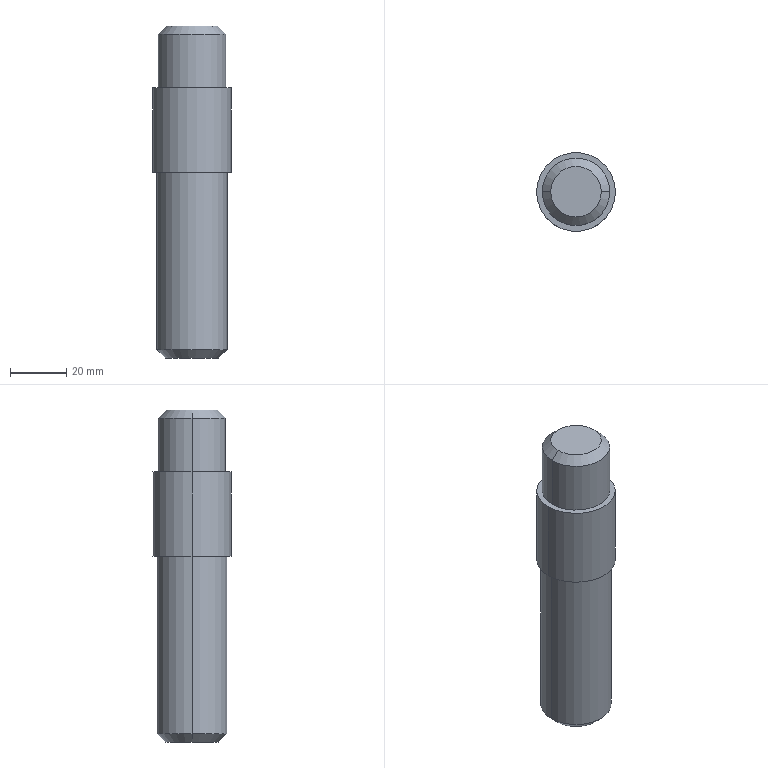Component | SolidWorks | PolishingAxis-1 | 1 solid | 14 faces | box 28 x 28 x 118 mm | volume 60187 mm3 | cylinder 6 | cone 4 | plane 4 | commonest cylinder face diameters 25 x2 24 x2 28 x2
build123d program:
from build123d import *

# Parameters (mm, degrees)
SKETCH1_R           = 12
BOSS_EXTRUDE1_DEPTH = 22
SKETCH2_R           = 14
BOSS_EXTRUDE2_DEPTH = 96
CUT_EXTRUDE1_START  = -66
SKETCH3_R           = 14
SKETCH3_R_2         = 12.5
CUT_EXTRUDE1_DEPTH  = 66
CHAMFER1_SIZE       = 3


with BuildPart() as part:
    # Sketch1 → Boss-Extrude1 (new body)
    with BuildSketch(Plane.XY):
        Circle(SKETCH1_R)
    extrude(amount=-BOSS_EXTRUDE1_DEPTH)

    # Sketch2 → Boss-Extrude2 (add)
    with BuildSketch(Plane.XY):
        Circle(SKETCH2_R)
    extrude(amount=BOSS_EXTRUDE2_DEPTH)

    # Sketch3 → Cut-Extrude1 (cut)
    with BuildSketch(Plane.XY.offset(96).offset(CUT_EXTRUDE1_START)):
        Circle(SKETCH3_R)
        Circle(SKETCH3_R_2, mode=Mode.SUBTRACT)
    extrude(amount=CUT_EXTRUDE1_DEPTH, mode=Mode.SUBTRACT)

    # Chamfer1
    chamfer1_edges = [part.edges().sort_by_distance(p)[0] for p in [
        (-12.5, 0, 96),
        (-12, 0, -22),
    ]]
    chamfer(chamfer1_edges, length=CHAMFER1_SIZE)


solid = part.part

# Placed as in the assembly
solid = solid.moved(Location((0, 0, -116), (180, 0, 0)))
STEP:
#1=COLOUR_RGB('',0.7922,0.8196,0.9333);
#2=FILL_AREA_STYLE_COLOUR('',#1);
#3=FILL_AREA_STYLE('',(#2));
#4=SURFACE_STYLE_FILL_AREA(#3);
#5=SURFACE_SIDE_STYLE('',(#4));
#6=SURFACE_STYLE_USAGE(.BOTH.,#5);
#7=PRESENTATION_STYLE_ASSIGNMENT((#6));
#8=CARTESIAN_POINT('',(-0.374,0.,-8.346));
#9=VERTEX_POINT('',#8);
#10=CARTESIAN_POINT('',(0.374,0.,-8.346));
#11=VERTEX_POINT('',#10);
#12=CARTESIAN_POINT('',(0.,0.,-8.346));
#13=DIRECTION('',(0.,0.,-1.));
#14=DIRECTION('',(-1.,0.,0.));
#15=AXIS2_PLACEMENT_3D('',#12,#13,#14);
#16=CIRCLE('',#15,0.374);
#17=EDGE_CURVE('',#9,#11,#16,.T.);
#18=ORIENTED_EDGE('',*,*,#17,.F.);
#19=CARTESIAN_POINT('',(-0.4921,0.,-8.228));
#20=VERTEX_POINT('',#19);
#21=CARTESIAN_POINT('',(-0.374,0.,-8.346));
#22=DIRECTION('',(-0.7071,0.,0.7071));
#23=VECTOR('',#22,39.37);
#24=LINE('',#21,#23);
#25=EDGE_CURVE('',#9,#20,#24,.T.);
#26=ORIENTED_EDGE('',*,*,#25,.T.);
#27=CARTESIAN_POINT('',(0.4921,0.,-8.228));
#28=VERTEX_POINT('',#27);
#29=CARTESIAN_POINT('',(0.,0.,-8.228));
#30=DIRECTION('',(0.,0.,1.));
#31=DIRECTION('',(-1.,0.,0.));
#32=AXIS2_PLACEMENT_3D('',#29,#30,#31);
#33=CIRCLE('',#32,0.4921);
#34=EDGE_CURVE('',#28,#20,#33,.T.);
#35=ORIENTED_EDGE('',*,*,#34,.F.);
#36=CARTESIAN_POINT('',(0.374,0.,-8.346));
#37=DIRECTION('',(0.7071,0.,0.7071));
#38=VECTOR('',#37,39.37);
#39=LINE('',#36,#38);
#40=EDGE_CURVE('',#11,#28,#39,.T.);
#41=ORIENTED_EDGE('',*,*,#40,.F.);
#42=EDGE_LOOP('',(#18,#26,#35,#41));
#43=FACE_OUTER_BOUND('',#42,.T.);
#44=CARTESIAN_POINT('',(0.,0.,-8.346));
#45=DIRECTION('',(0.,0.,1.));
#46=DIRECTION('',(1.,0.,0.));
#47=AXIS2_PLACEMENT_3D('',#44,#45,#46);
#48=CONICAL_SURFACE('',#47,0.374,0.7854);
#49=ADVANCED_FACE('',(#43),#48,.T.);
#50=CARTESIAN_POINT('',(0.3543,0.,-3.701));
#51=VERTEX_POINT('',#50);
#52=CARTESIAN_POINT('',(-0.3543,0.,-3.701));
#53=VERTEX_POINT('',#52);
#54=CARTESIAN_POINT('',(0.,0.,-3.701));
#55=DIRECTION('',(0.,0.,1.));
#56=DIRECTION('',(-1.,0.,0.));
#57=AXIS2_PLACEMENT_3D('',#54,#55,#56);
#58=CIRCLE('',#57,0.3543);
#59=EDGE_CURVE('',#51,#53,#58,.T.);
#60=ORIENTED_EDGE('',*,*,#59,.F.);
#61=CARTESIAN_POINT('',(0.4724,0.,-3.819));
#62=VERTEX_POINT('',#61);
#63=CARTESIAN_POINT('',(0.4724,0.,-3.819));
#64=DIRECTION('',(0.7071,0.,-0.7071));
#65=VECTOR('',#64,39.37);
#66=LINE('',#63,#65);
#67=EDGE_CURVE('',#51,#62,#66,.T.);
#68=ORIENTED_EDGE('',*,*,#67,.T.);
#69=CARTESIAN_POINT('',(-0.4724,0.,-3.819));
#70=VERTEX_POINT('',#69);
#71=CARTESIAN_POINT('',(0.,0.,-3.819));
#72=DIRECTION('',(0.,0.,-1.));
#73=DIRECTION('',(-1.,0.,0.));
#74=AXIS2_PLACEMENT_3D('',#71,#72,#73);
#75=CIRCLE('',#74,0.4724);
#76=EDGE_CURVE('',#70,#62,#75,.T.);
#77=ORIENTED_EDGE('',*,*,#76,.F.);
#78=CARTESIAN_POINT('',(-0.4724,0.,-3.819));
#79=DIRECTION('',(-0.7071,0.,-0.7071));
#80=VECTOR('',#79,39.37);
#81=LINE('',#78,#80);
#82=EDGE_CURVE('',#53,#70,#81,.T.);
#83=ORIENTED_EDGE('',*,*,#82,.F.);
#84=EDGE_LOOP('',(#60,#68,#77,#83));
#85=FACE_OUTER_BOUND('',#84,.T.);
#86=CARTESIAN_POINT('',(0.,0.,-3.819));
#87=DIRECTION('',(0.,0.,-1.));
#88=DIRECTION('',(-1.,0.,0.));
#89=AXIS2_PLACEMENT_3D('',#86,#87,#88);
#90=CONICAL_SURFACE('',#89,0.4724,0.7854);
#91=ADVANCED_FACE('',(#85),#90,.T.);
#92=CARTESIAN_POINT('',(-0.4921,0.,-5.748));
#93=VERTEX_POINT('',#92);
#94=CARTESIAN_POINT('',(0.4921,0.,-5.748));
#95=VERTEX_POINT('',#94);
#96=CARTESIAN_POINT('',(0.,0.,-5.748));
#97=DIRECTION('',(0.,0.,-1.));
#98=DIRECTION('',(-1.,0.,0.));
#99=AXIS2_PLACEMENT_3D('',#96,#97,#98);
#100=CIRCLE('',#99,0.4921);
#101=EDGE_CURVE('',#93,#95,#100,.T.);
#102=ORIENTED_EDGE('',*,*,#101,.T.);
#103=CARTESIAN_POINT('',(0.4921,0.,-5.748));
#104=DIRECTION('',(0.,0.,-1.));
#105=VECTOR('',#104,39.37);
#106=LINE('',#103,#105);
#107=EDGE_CURVE('',#95,#28,#106,.T.);
#108=ORIENTED_EDGE('',*,*,#107,.T.);
#109=ORIENTED_EDGE('',*,*,#34,.T.);
#110=CARTESIAN_POINT('',(-0.4921,0.,-5.748));
#111=DIRECTION('',(0.,0.,-1.));
#112=VECTOR('',#111,39.37);
#113=LINE('',#110,#112);
#114=EDGE_CURVE('',#93,#20,#113,.T.);
#115=ORIENTED_EDGE('',*,*,#114,.F.);
#116=EDGE_LOOP('',(#102,#108,#109,#115));
#117=FACE_OUTER_BOUND('',#116,.T.);
#118=CARTESIAN_POINT('',(0.,0.,-5.748));
#119=DIRECTION('',(0.,0.,-1.));
#120=DIRECTION('',(-1.,0.,0.));
#121=AXIS2_PLACEMENT_3D('',#118,#119,#120);
#122=CYLINDRICAL_SURFACE('',#121,0.4921);
#123=ADVANCED_FACE('',(#117),#122,.T.);
#124=ORIENTED_EDGE('',*,*,#76,.T.);
#125=CARTESIAN_POINT('',(0.4724,0.,-4.567));
#126=VERTEX_POINT('',#125);
#127=CARTESIAN_POINT('',(0.4724,0.,-3.701));
#128=DIRECTION('',(0.,0.,-1.));
#129=VECTOR('',#128,39.37);
#130=LINE('',#127,#129);
#131=EDGE_CURVE('',#62,#126,#130,.T.);
#132=ORIENTED_EDGE('',*,*,#131,.T.);
#133=CARTESIAN_POINT('',(-0.4724,0.,-4.567));
#134=VERTEX_POINT('',#133);
#135=CARTESIAN_POINT('',(0.,0.,-4.567));
#136=DIRECTION('',(0.,0.,-1.));
#137=DIRECTION('',(-1.,0.,0.));
#138=AXIS2_PLACEMENT_3D('',#135,#136,#137);
#139=CIRCLE('',#138,0.4724);
#140=EDGE_CURVE('',#134,#126,#139,.T.);
#141=ORIENTED_EDGE('',*,*,#140,.F.);
#142=CARTESIAN_POINT('',(-0.4724,0.,-3.701));
#143=DIRECTION('',(0.,0.,-1.));
#144=VECTOR('',#143,39.37);
#145=LINE('',#142,#144);
#146=EDGE_CURVE('',#70,#134,#145,.T.);
#147=ORIENTED_EDGE('',*,*,#146,.F.);
#148=EDGE_LOOP('',(#124,#132,#141,#147));
#149=FACE_OUTER_BOUND('',#148,.T.);
#150=CARTESIAN_POINT('',(0.,0.,-3.701));
#151=DIRECTION('',(0.,0.,-1.));
#152=DIRECTION('',(-1.,0.,0.));
#153=AXIS2_PLACEMENT_3D('',#150,#151,#152);
#154=CYLINDRICAL_SURFACE('',#153,0.4724);
#155=ADVANCED_FACE('',(#149),#154,.T.);
#156=CARTESIAN_POINT('',(-0.5512,0.,-5.748));
#157=VERTEX_POINT('',#156);
#158=CARTESIAN_POINT('',(0.5512,0.,-5.748));
#159=VERTEX_POINT('',#158);
#160=CARTESIAN_POINT('',(0.,0.,-5.748));
#161=DIRECTION('',(0.,0.,-1.));
#162=DIRECTION('',(-1.,0.,0.));
#163=AXIS2_PLACEMENT_3D('',#160,#161,#162);
#164=CIRCLE('',#163,0.5512);
#165=EDGE_CURVE('',#157,#159,#164,.T.);
#166=ORIENTED_EDGE('',*,*,#165,.F.);
#167=CARTESIAN_POINT('',(-0.5512,0.,-4.567));
#168=VERTEX_POINT('',#167);
#169=CARTESIAN_POINT('',(-0.5512,0.,-8.346));
#170=DIRECTION('',(0.,0.,1.));
#171=VECTOR('',#170,39.37);
#172=LINE('',#169,#171);
#173=EDGE_CURVE('',#157,#168,#172,.T.);
#174=ORIENTED_EDGE('',*,*,#173,.T.);
#175=CARTESIAN_POINT('',(0.5512,0.,-4.567));
#176=VERTEX_POINT('',#175);
#177=CARTESIAN_POINT('',(0.,0.,-4.567));
#178=DIRECTION('',(0.,0.,-1.));
#179=DIRECTION('',(-1.,0.,0.));
#180=AXIS2_PLACEMENT_3D('',#177,#178,#179);
#181=CIRCLE('',#180,0.5512);
#182=EDGE_CURVE('',#168,#176,#181,.T.);
#183=ORIENTED_EDGE('',*,*,#182,.T.);
#184=CARTESIAN_POINT('',(0.5512,0.,-8.346));
#185=DIRECTION('',(0.,0.,1.));
#186=VECTOR('',#185,39.37);
#187=LINE('',#184,#186);
#188=EDGE_CURVE('',#159,#176,#187,.T.);
#189=ORIENTED_EDGE('',*,*,#188,.F.);
#190=EDGE_LOOP('',(#166,#174,#183,#189));
#191=FACE_OUTER_BOUND('',#190,.T.);
#192=CARTESIAN_POINT('',(0.,0.,-8.346));
#193=DIRECTION('',(0.,0.,1.));
#194=DIRECTION('',(1.,0.,0.));
#195=AXIS2_PLACEMENT_3D('',#192,#193,#194);
#196=CYLINDRICAL_SURFACE('',#195,0.5512);
#197=ADVANCED_FACE('',(#191),#196,.T.);
#198=ORIENTED_EDGE('',*,*,#173,.F.);
#199=CARTESIAN_POINT('',(0.,0.,-5.748));
#200=DIRECTION('',(0.,0.,-1.));
#201=DIRECTION('',(-1.,0.,0.));
#202=AXIS2_PLACEMENT_3D('',#199,#200,#201);
#203=CIRCLE('',#202,0.5512);
#204=EDGE_CURVE('',#159,#157,#203,.T.);
#205=ORIENTED_EDGE('',*,*,#204,.F.);
#206=ORIENTED_EDGE('',*,*,#188,.T.);
#207=CARTESIAN_POINT('',(0.,0.,-4.567));
#208=DIRECTION('',(0.,0.,-1.));
#209=DIRECTION('',(-1.,0.,0.));
#210=AXIS2_PLACEMENT_3D('',#207,#208,#209);
#211=CIRCLE('',#210,0.5512);
#212=EDGE_CURVE('',#176,#168,#211,.T.);
#213=ORIENTED_EDGE('',*,*,#212,.T.);
#214=EDGE_LOOP('',(#198,#205,#206,#213));
#215=FACE_OUTER_BOUND('',#214,.T.);
#216=CARTESIAN_POINT('',(0.,0.,-8.346));
#217=DIRECTION('',(0.,0.,1.));
#218=DIRECTION('',(1.,0.,0.));
#219=AXIS2_PLACEMENT_3D('',#216,#217,#218);
#220=CYLINDRICAL_SURFACE('',#219,0.5512);
#221=ADVANCED_FACE('',(#215),#220,.T.);
#222=ORIENTED_EDGE('',*,*,#131,.F.);
#223=CARTESIAN_POINT('',(0.,0.,-3.819));
#224=DIRECTION('',(0.,0.,-1.));
#225=DIRECTION('',(-1.,0.,0.));
#226=AXIS2_PLACEMENT_3D('',#223,#224,#225);
#227=CIRCLE('',#226,0.4724);
#228=EDGE_CURVE('',#62,#70,#227,.T.);
#229=ORIENTED_EDGE('',*,*,#228,.T.);
#230=ORIENTED_EDGE('',*,*,#146,.T.);
#231=CARTESIAN_POINT('',(0.,0.,-4.567));
#232=DIRECTION('',(0.,0.,-1.));
#233=DIRECTION('',(-1.,0.,0.));
#234=AXIS2_PLACEMENT_3D('',#231,#232,#233);
#235=CIRCLE('',#234,0.4724);
#236=EDGE_CURVE('',#126,#134,#235,.T.);
#237=ORIENTED_EDGE('',*,*,#236,.F.);
#238=EDGE_LOOP('',(#222,#229,#230,#237));
#239=FACE_OUTER_BOUND('',#238,.T.);
#240=CARTESIAN_POINT('',(0.,0.,-3.701));
#241=DIRECTION('',(0.,0.,-1.));
#242=DIRECTION('',(-1.,0.,0.));
#243=AXIS2_PLACEMENT_3D('',#240,#241,#242);
#244=CYLINDRICAL_SURFACE('',#243,0.4724);
#245=ADVANCED_FACE('',(#239),#244,.T.);
#246=CARTESIAN_POINT('',(0.,0.,-3.701));
#247=DIRECTION('',(0.,0.,1.));
#248=DIRECTION('',(-1.,0.,0.));
#249=AXIS2_PLACEMENT_3D('',#246,#247,#248);
#250=CIRCLE('',#249,0.3543);
#251=EDGE_CURVE('',#53,#51,#250,.T.);
#252=ORIENTED_EDGE('',*,*,#251,.T.);
#253=ORIENTED_EDGE('',*,*,#59,.T.);
#254=EDGE_LOOP('',(#252,#253));
#255=FACE_OUTER_BOUND('',#254,.T.);
#256=CARTESIAN_POINT('',(0.,0.,-3.701));
#257=DIRECTION('',(0.,0.,-1.));
#258=DIRECTION('',(-1.,0.,0.));
#259=AXIS2_PLACEMENT_3D('',#256,#257,#258);
#260=PLANE('',#259);
#261=ADVANCED_FACE('',(#255),#260,.F.);
#262=ORIENTED_EDGE('',*,*,#140,.T.);
#263=ORIENTED_EDGE('',*,*,#236,.T.);
#264=EDGE_LOOP('',(#262,#263));
#265=FACE_BOUND('',#264,.T.);
#266=ORIENTED_EDGE('',*,*,#212,.F.);
#267=ORIENTED_EDGE('',*,*,#182,.F.);
#268=EDGE_LOOP('',(#266,#267));
#269=FACE_OUTER_BOUND('',#268,.T.);
#270=CARTESIAN_POINT('',(0.,0.,-4.567));
#271=DIRECTION('',(0.,0.,-1.));
#272=DIRECTION('',(-1.,0.,0.));
#273=AXIS2_PLACEMENT_3D('',#270,#271,#272);
#274=PLANE('',#273);
#275=ADVANCED_FACE('',(#265,#269),#274,.F.);
#276=ORIENTED_EDGE('',*,*,#101,.F.);
#277=CARTESIAN_POINT('',(0.,0.,-5.748));
#278=DIRECTION('',(0.,0.,-1.));
#279=DIRECTION('',(-1.,0.,0.));
#280=AXIS2_PLACEMENT_3D('',#277,#278,#279);
#281=CIRCLE('',#280,0.4921);
#282=EDGE_CURVE('',#95,#93,#281,.T.);
#283=ORIENTED_EDGE('',*,*,#282,.F.);
#284=EDGE_LOOP('',(#276,#283));
#285=FACE_BOUND('',#284,.T.);
#286=ORIENTED_EDGE('',*,*,#204,.T.);
#287=ORIENTED_EDGE('',*,*,#165,.T.);
#288=EDGE_LOOP('',(#286,#287));
#289=FACE_OUTER_BOUND('',#288,.T.);
#290=CARTESIAN_POINT('',(0.,0.,-5.748));
#291=DIRECTION('',(0.,0.,-1.));
#292=DIRECTION('',(-1.,0.,0.));
#293=AXIS2_PLACEMENT_3D('',#290,#291,#292);
#294=PLANE('',#293);
#295=ADVANCED_FACE('',(#285,#289),#294,.T.);
#296=ORIENTED_EDGE('',*,*,#107,.F.);
#297=ORIENTED_EDGE('',*,*,#282,.T.);
#298=ORIENTED_EDGE('',*,*,#114,.T.);
#299=CARTESIAN_POINT('',(0.,0.,-8.228));
#300=DIRECTION('',(0.,0.,1.));
#301=DIRECTION('',(-1.,0.,0.));
#302=AXIS2_PLACEMENT_3D('',#299,#300,#301);
#303=CIRCLE('',#302,0.4921);
#304=EDGE_CURVE('',#20,#28,#303,.T.);
#305=ORIENTED_EDGE('',*,*,#304,.T.);
#306=EDGE_LOOP('',(#296,#297,#298,#305));
#307=FACE_OUTER_BOUND('',#306,.T.);
#308=CARTESIAN_POINT('',(0.,0.,-5.748));
#309=DIRECTION('',(0.,0.,-1.));
#310=DIRECTION('',(-1.,0.,0.));
#311=AXIS2_PLACEMENT_3D('',#308,#309,#310);
#312=CYLINDRICAL_SURFACE('',#311,0.4921);
#313=ADVANCED_FACE('',(#307),#312,.T.);
#314=CARTESIAN_POINT('',(0.,0.,-8.346));
#315=DIRECTION('',(0.,0.,-1.));
#316=DIRECTION('',(-1.,0.,0.));
#317=AXIS2_PLACEMENT_3D('',#314,#315,#316);
#318=CIRCLE('',#317,0.374);
#319=EDGE_CURVE('',#11,#9,#318,.T.);
#320=ORIENTED_EDGE('',*,*,#319,.T.);
#321=ORIENTED_EDGE('',*,*,#17,.T.);
#322=EDGE_LOOP('',(#320,#321));
#323=FACE_OUTER_BOUND('',#322,.T.);
#324=CARTESIAN_POINT('',(0.,0.,-8.346));
#325=DIRECTION('',(0.,0.,-1.));
#326=DIRECTION('',(-1.,0.,0.));
#327=AXIS2_PLACEMENT_3D('',#324,#325,#326);
#328=PLANE('',#327);
#329=ADVANCED_FACE('',(#323),#328,.T.);
#330=ORIENTED_EDGE('',*,*,#67,.F.);
#331=ORIENTED_EDGE('',*,*,#251,.F.);
#332=ORIENTED_EDGE('',*,*,#82,.T.);
#333=ORIENTED_EDGE('',*,*,#228,.F.);
#334=EDGE_LOOP('',(#330,#331,#332,#333));
#335=FACE_OUTER_BOUND('',#334,.T.);
#336=CARTESIAN_POINT('',(0.,0.,-3.819));
#337=DIRECTION('',(0.,0.,-1.));
#338=DIRECTION('',(-1.,0.,0.));
#339=AXIS2_PLACEMENT_3D('',#336,#337,#338);
#340=CONICAL_SURFACE('',#339,0.4724,0.7854);
#341=ADVANCED_FACE('',(#335),#340,.T.);
#342=ORIENTED_EDGE('',*,*,#25,.F.);
#343=ORIENTED_EDGE('',*,*,#319,.F.);
#344=ORIENTED_EDGE('',*,*,#40,.T.);
#345=ORIENTED_EDGE('',*,*,#304,.F.);
#346=EDGE_LOOP('',(#342,#343,#344,#345));
#347=FACE_OUTER_BOUND('',#346,.T.);
#348=CARTESIAN_POINT('',(0.,0.,-8.346));
#349=DIRECTION('',(0.,0.,1.));
#350=DIRECTION('',(1.,0.,0.));
#351=AXIS2_PLACEMENT_3D('',#348,#349,#350);
#352=CONICAL_SURFACE('',#351,0.374,0.7854);
#353=ADVANCED_FACE('',(#347),#352,.T.);
#354=CLOSED_SHELL('',(#49,#91,#123,#155,#197,#221,#245,#261,#275,#295,#313,#329,#341,#353));
#355=MANIFOLD_SOLID_BREP('',#354);
#356=STYLED_ITEM('',(#7),#355);
#357=(LENGTH_UNIT()NAMED_UNIT(*)SI_UNIT($,.METRE.));
#358=LENGTH_MEASURE_WITH_UNIT(LENGTH_MEASURE(0.0254),#357);
#359=DIMENSIONAL_EXPONENTS(1.,0.,0.,0.,0.,0.,0.);
#360=(CONVERSION_BASED_UNIT('',#358)LENGTH_UNIT()NAMED_UNIT(#359));
#361=UNCERTAINTY_MEASURE_WITH_UNIT(LENGTH_MEASURE(0.00001),#360,'','');
#362=(NAMED_UNIT(*)PLANE_ANGLE_UNIT()SI_UNIT($,.RADIAN.));
#363=(NAMED_UNIT(*)SI_UNIT($,.STERADIAN.)SOLID_ANGLE_UNIT());
#364=(GEOMETRIC_REPRESENTATION_CONTEXT(3)GLOBAL_UNCERTAINTY_ASSIGNED_CONTEXT((#361))GLOBAL_UNIT_ASSIGNED_CONTEXT((#360,#362,#363))REPRESENTATION_CONTEXT('',''));
#365=MECHANICAL_DESIGN_GEOMETRIC_PRESENTATION_REPRESENTATION('',(#356),#364);
#366=CARTESIAN_POINT('',(0.,0.,0.));
#367=DIRECTION('',(0.,0.,1.));
#368=DIRECTION('',(1.,0.,0.));
#369=AXIS2_PLACEMENT_3D('',#366,#367,#368);
#370=(LENGTH_UNIT()NAMED_UNIT(*)SI_UNIT($,.METRE.));
#371=LENGTH_MEASURE_WITH_UNIT(LENGTH_MEASURE(0.0254),#370);
#372=DIMENSIONAL_EXPONENTS(1.,0.,0.,0.,0.,0.,0.);
#373=(CONVERSION_BASED_UNIT('',#371)LENGTH_UNIT()NAMED_UNIT(#372));
#374=UNCERTAINTY_MEASURE_WITH_UNIT(LENGTH_MEASURE(0.00001),#373,'','');
#375=(NAMED_UNIT(*)PLANE_ANGLE_UNIT()SI_UNIT($,.RADIAN.));
#376=(NAMED_UNIT(*)SI_UNIT($,.STERADIAN.)SOLID_ANGLE_UNIT());
#377=(GEOMETRIC_REPRESENTATION_CONTEXT(3)GLOBAL_UNCERTAINTY_ASSIGNED_CONTEXT((#374))GLOBAL_UNIT_ASSIGNED_CONTEXT((#373,#375,#376))REPRESENTATION_CONTEXT('',''));
#378=ADVANCED_BREP_SHAPE_REPRESENTATION('',(#355,#369),#377);
#379=PRESENTATION_LAYER_ASSIGNMENT('','',(#356));